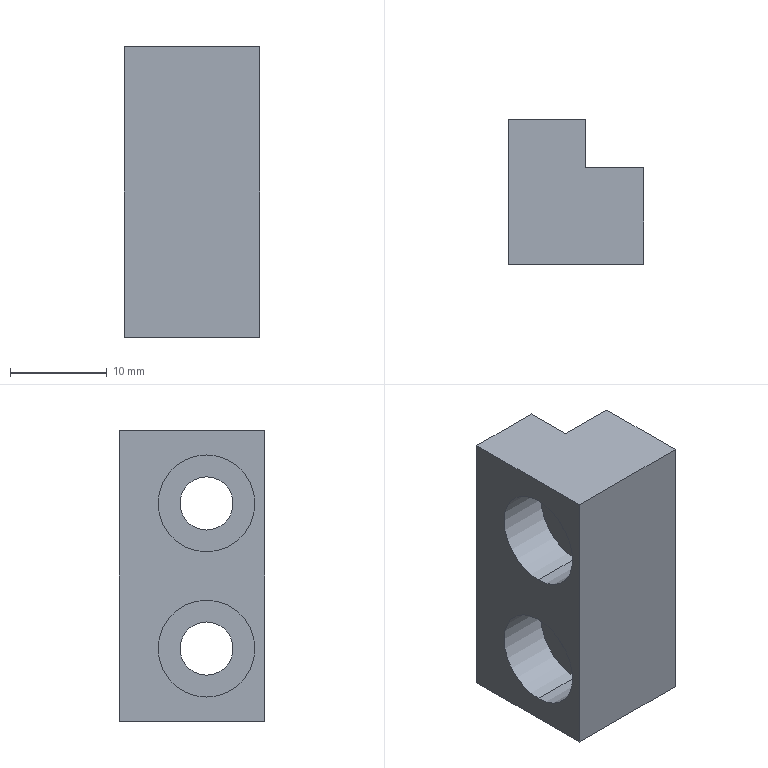Component | SolidWorks | 8TC-A15004-60-34B-1 | 1 solid | 18 faces | box 14 x 15 x 30 mm | volume 4143 mm3 | plane 10 | cylinder 8 | commonest cylinder face diameters 10 x4 5.5 x4 | material #45
build123d program:
from build123d import *

# Parameters (mm, degrees)
SKETCH1_W                                       = 15
SKETCH1_H                                       = 30
BOSS_EXTRUDE1_DEPTH                             = 7
SKETCH2_W                                       = 5
SKETCH2_H                                       = 6
CUT_EXTRUDE1_DEPTH                              = 32.706
M5_HEX_SOCKET_HEAD_CAP_SCREW_CBORE1_D           = 5.5
M5_HEX_SOCKET_HEAD_CAP_SCREW_CBORE1_CBORE_D     = 10
M5_HEX_SOCKET_HEAD_CAP_SCREW_CBORE1_CBORE_DEPTH = 5.4


with BuildPart() as part:
    # Sketch1 → Boss-Extrude1 (new, symmetric)
    with BuildSketch(Plane(origin=(0, 0, 0), x_dir=(1, 0, 0), z_dir=(0, 1, 0))):
        Rectangle(SKETCH1_W, SKETCH1_H)
    extrude(amount=BOSS_EXTRUDE1_DEPTH, both=True)

    # Sketch2 → Cut-Extrude1 (cut, through all)
    with BuildSketch(Plane.XY.offset(15)):
        with Locations((-5, -4)):
            Rectangle(SKETCH2_W, SKETCH2_H)
    extrude(amount=-CUT_EXTRUDE1_DEPTH, mode=Mode.SUBTRACT)

    # M5 Hex Socket Head Cap Screw CBORE1 (through all)
    with Locations(Plane(origin=(0, 7, 0), x_dir=(1, 0, 0), z_dir=(0, 1, 0))):
        with Locations((1.5, 7.5), (1.5, -7.5)):
            CounterBoreHole(M5_HEX_SOCKET_HEAD_CAP_SCREW_CBORE1_D / 2, M5_HEX_SOCKET_HEAD_CAP_SCREW_CBORE1_CBORE_D / 2, M5_HEX_SOCKET_HEAD_CAP_SCREW_CBORE1_CBORE_DEPTH)


solid = part.part

# Placed as in the assembly
solid = solid.moved(Location((-104.286, -69.5, 0), (180, 0, 90)))
STEP:
#1=COLOUR_RGB('',0.7922,0.8196,0.9333);
#2=FILL_AREA_STYLE_COLOUR('',#1);
#3=FILL_AREA_STYLE('',(#2));
#4=SURFACE_STYLE_FILL_AREA(#3);
#5=SURFACE_SIDE_STYLE('',(#4));
#6=SURFACE_STYLE_USAGE(.BOTH.,#5);
#7=PRESENTATION_STYLE_ASSIGNMENT((#6));
#8=CARTESIAN_POINT('',(-4.169,-2.795,0.4921));
#9=VERTEX_POINT('',#8);
#10=CARTESIAN_POINT('',(-4.169,-2.795,0.09843));
#11=VERTEX_POINT('',#10);
#12=CARTESIAN_POINT('',(-4.169,-2.795,0.2953));
#13=DIRECTION('',(-1.,0.,0.));
#14=DIRECTION('',(0.,0.,-1.));
#15=AXIS2_PLACEMENT_3D('',#12,#13,#14);
#16=CIRCLE('',#15,0.1969);
#17=EDGE_CURVE('',#9,#11,#16,.T.);
#18=ORIENTED_EDGE('',*,*,#17,.F.);
#19=CARTESIAN_POINT('',(-4.381,-2.795,0.4921));
#20=VERTEX_POINT('',#19);
#21=CARTESIAN_POINT('',(-4.381,-2.795,0.4921));
#22=DIRECTION('',(-1.,0.,0.));
#23=VECTOR('',#22,39.37);
#24=LINE('',#21,#23);
#25=EDGE_CURVE('',#9,#20,#24,.T.);
#26=ORIENTED_EDGE('',*,*,#25,.T.);
#27=CARTESIAN_POINT('',(-4.381,-2.795,0.09843));
#28=VERTEX_POINT('',#27);
#29=CARTESIAN_POINT('',(-4.381,-2.795,0.2953));
#30=DIRECTION('',(-1.,0.,0.));
#31=DIRECTION('',(0.,0.,-1.));
#32=AXIS2_PLACEMENT_3D('',#29,#30,#31);
#33=CIRCLE('',#32,0.1969);
#34=EDGE_CURVE('',#20,#28,#33,.T.);
#35=ORIENTED_EDGE('',*,*,#34,.T.);
#36=CARTESIAN_POINT('',(-4.381,-2.795,0.09843));
#37=DIRECTION('',(-1.,0.,0.));
#38=VECTOR('',#37,39.37);
#39=LINE('',#36,#38);
#40=EDGE_CURVE('',#11,#28,#39,.T.);
#41=ORIENTED_EDGE('',*,*,#40,.F.);
#42=EDGE_LOOP('',(#18,#26,#35,#41));
#43=FACE_OUTER_BOUND('',#42,.T.);
#44=CARTESIAN_POINT('',(-4.381,-2.795,0.2953));
#45=DIRECTION('',(-1.,0.,0.));
#46=DIRECTION('',(0.,0.,-1.));
#47=AXIS2_PLACEMENT_3D('',#44,#45,#46);
#48=CYLINDRICAL_SURFACE('',#47,0.1969);
#49=ADVANCED_FACE('',(#43),#48,.F.);
#50=CARTESIAN_POINT('',(-3.83,-2.795,0.4035));
#51=VERTEX_POINT('',#50);
#52=CARTESIAN_POINT('',(-3.83,-2.795,0.187));
#53=VERTEX_POINT('',#52);
#54=CARTESIAN_POINT('',(-3.83,-2.795,0.2953));
#55=DIRECTION('',(-1.,0.,0.));
#56=DIRECTION('',(0.,0.,-1.));
#57=AXIS2_PLACEMENT_3D('',#54,#55,#56);
#58=CIRCLE('',#57,0.1083);
#59=EDGE_CURVE('',#51,#53,#58,.T.);
#60=ORIENTED_EDGE('',*,*,#59,.F.);
#61=CARTESIAN_POINT('',(-4.169,-2.795,0.4035));
#62=VERTEX_POINT('',#61);
#63=CARTESIAN_POINT('',(-4.381,-2.795,0.4035));
#64=DIRECTION('',(-1.,0.,0.));
#65=VECTOR('',#64,39.37);
#66=LINE('',#63,#65);
#67=EDGE_CURVE('',#51,#62,#66,.T.);
#68=ORIENTED_EDGE('',*,*,#67,.T.);
#69=CARTESIAN_POINT('',(-4.169,-2.795,0.187));
#70=VERTEX_POINT('',#69);
#71=CARTESIAN_POINT('',(-4.169,-2.795,0.2953));
#72=DIRECTION('',(-1.,0.,0.));
#73=DIRECTION('',(0.,0.,-1.));
#74=AXIS2_PLACEMENT_3D('',#71,#72,#73);
#75=CIRCLE('',#74,0.1083);
#76=EDGE_CURVE('',#62,#70,#75,.T.);
#77=ORIENTED_EDGE('',*,*,#76,.T.);
#78=CARTESIAN_POINT('',(-4.381,-2.795,0.187));
#79=DIRECTION('',(-1.,0.,0.));
#80=VECTOR('',#79,39.37);
#81=LINE('',#78,#80);
#82=EDGE_CURVE('',#53,#70,#81,.T.);
#83=ORIENTED_EDGE('',*,*,#82,.F.);
#84=EDGE_LOOP('',(#60,#68,#77,#83));
#85=FACE_OUTER_BOUND('',#84,.T.);
#86=CARTESIAN_POINT('',(-4.381,-2.795,0.2953));
#87=DIRECTION('',(-1.,0.,0.));
#88=DIRECTION('',(0.,0.,-1.));
#89=AXIS2_PLACEMENT_3D('',#86,#87,#88);
#90=CYLINDRICAL_SURFACE('',#89,0.1083);
#91=ADVANCED_FACE('',(#85),#90,.F.);
#92=CARTESIAN_POINT('',(-4.169,-2.795,-0.09843));
#93=VERTEX_POINT('',#92);
#94=CARTESIAN_POINT('',(-4.169,-2.795,-0.4921));
#95=VERTEX_POINT('',#94);
#96=CARTESIAN_POINT('',(-4.169,-2.795,-0.2953));
#97=DIRECTION('',(-1.,0.,0.));
#98=DIRECTION('',(0.,0.,-1.));
#99=AXIS2_PLACEMENT_3D('',#96,#97,#98);
#100=CIRCLE('',#99,0.1969);
#101=EDGE_CURVE('',#93,#95,#100,.T.);
#102=ORIENTED_EDGE('',*,*,#101,.F.);
#103=CARTESIAN_POINT('',(-4.381,-2.795,-0.09843));
#104=VERTEX_POINT('',#103);
#105=CARTESIAN_POINT('',(-4.381,-2.795,-0.09843));
#106=DIRECTION('',(-1.,0.,0.));
#107=VECTOR('',#106,39.37);
#108=LINE('',#105,#107);
#109=EDGE_CURVE('',#93,#104,#108,.T.);
#110=ORIENTED_EDGE('',*,*,#109,.T.);
#111=CARTESIAN_POINT('',(-4.381,-2.795,-0.4921));
#112=VERTEX_POINT('',#111);
#113=CARTESIAN_POINT('',(-4.381,-2.795,-0.2953));
#114=DIRECTION('',(-1.,0.,0.));
#115=DIRECTION('',(0.,0.,-1.));
#116=AXIS2_PLACEMENT_3D('',#113,#114,#115);
#117=CIRCLE('',#116,0.1969);
#118=EDGE_CURVE('',#104,#112,#117,.T.);
#119=ORIENTED_EDGE('',*,*,#118,.T.);
#120=CARTESIAN_POINT('',(-4.381,-2.795,-0.4921));
#121=DIRECTION('',(-1.,0.,0.));
#122=VECTOR('',#121,39.37);
#123=LINE('',#120,#122);
#124=EDGE_CURVE('',#95,#112,#123,.T.);
#125=ORIENTED_EDGE('',*,*,#124,.F.);
#126=EDGE_LOOP('',(#102,#110,#119,#125));
#127=FACE_OUTER_BOUND('',#126,.T.);
#128=CARTESIAN_POINT('',(-4.381,-2.795,-0.2953));
#129=DIRECTION('',(-1.,0.,0.));
#130=DIRECTION('',(0.,0.,-1.));
#131=AXIS2_PLACEMENT_3D('',#128,#129,#130);
#132=CYLINDRICAL_SURFACE('',#131,0.1969);
#133=ADVANCED_FACE('',(#127),#132,.F.);
#134=CARTESIAN_POINT('',(-3.83,-2.795,-0.187));
#135=VERTEX_POINT('',#134);
#136=CARTESIAN_POINT('',(-3.83,-2.795,-0.4035));
#137=VERTEX_POINT('',#136);
#138=CARTESIAN_POINT('',(-3.83,-2.795,-0.2953));
#139=DIRECTION('',(-1.,0.,0.));
#140=DIRECTION('',(0.,0.,-1.));
#141=AXIS2_PLACEMENT_3D('',#138,#139,#140);
#142=CIRCLE('',#141,0.1083);
#143=EDGE_CURVE('',#135,#137,#142,.T.);
#144=ORIENTED_EDGE('',*,*,#143,.F.);
#145=CARTESIAN_POINT('',(-4.169,-2.795,-0.187));
#146=VERTEX_POINT('',#145);
#147=CARTESIAN_POINT('',(-4.381,-2.795,-0.187));
#148=DIRECTION('',(-1.,0.,0.));
#149=VECTOR('',#148,39.37);
#150=LINE('',#147,#149);
#151=EDGE_CURVE('',#135,#146,#150,.T.);
#152=ORIENTED_EDGE('',*,*,#151,.T.);
#153=CARTESIAN_POINT('',(-4.169,-2.795,-0.4035));
#154=VERTEX_POINT('',#153);
#155=CARTESIAN_POINT('',(-4.169,-2.795,-0.2953));
#156=DIRECTION('',(-1.,0.,0.));
#157=DIRECTION('',(0.,0.,-1.));
#158=AXIS2_PLACEMENT_3D('',#155,#156,#157);
#159=CIRCLE('',#158,0.1083);
#160=EDGE_CURVE('',#146,#154,#159,.T.);
#161=ORIENTED_EDGE('',*,*,#160,.T.);
#162=CARTESIAN_POINT('',(-4.381,-2.795,-0.4035));
#163=DIRECTION('',(-1.,0.,0.));
#164=VECTOR('',#163,39.37);
#165=LINE('',#162,#164);
#166=EDGE_CURVE('',#137,#154,#165,.T.);
#167=ORIENTED_EDGE('',*,*,#166,.F.);
#168=EDGE_LOOP('',(#144,#152,#161,#167));
#169=FACE_OUTER_BOUND('',#168,.T.);
#170=CARTESIAN_POINT('',(-4.381,-2.795,-0.2953));
#171=DIRECTION('',(-1.,0.,0.));
#172=DIRECTION('',(0.,0.,-1.));
#173=AXIS2_PLACEMENT_3D('',#170,#171,#172);
#174=CYLINDRICAL_SURFACE('',#173,0.1083);
#175=ADVANCED_FACE('',(#169),#174,.F.);
#176=CARTESIAN_POINT('',(-3.83,-2.638,0.5906));
#177=VERTEX_POINT('',#176);
#178=CARTESIAN_POINT('',(-3.83,-2.638,-0.5906));
#179=VERTEX_POINT('',#178);
#180=CARTESIAN_POINT('',(-3.83,-2.638,0.5906));
#181=DIRECTION('',(-0.,-0.,-1.));
#182=VECTOR('',#181,39.37);
#183=LINE('',#180,#182);
#184=EDGE_CURVE('',#177,#179,#183,.T.);
#185=ORIENTED_EDGE('',*,*,#184,.F.);
#186=CARTESIAN_POINT('',(-3.83,-3.031,0.5906));
#187=VERTEX_POINT('',#186);
#188=CARTESIAN_POINT('',(-3.83,-2.441,0.5906));
#189=DIRECTION('',(0.,1.,-0.));
#190=VECTOR('',#189,39.37);
#191=LINE('',#188,#190);
#192=EDGE_CURVE('',#187,#177,#191,.T.);
#193=ORIENTED_EDGE('',*,*,#192,.F.);
#194=CARTESIAN_POINT('',(-3.83,-3.031,-0.5906));
#195=VERTEX_POINT('',#194);
#196=CARTESIAN_POINT('',(-3.83,-3.031,-0.5906));
#197=DIRECTION('',(0.,0.,1.));
#198=VECTOR('',#197,39.37);
#199=LINE('',#196,#198);
#200=EDGE_CURVE('',#195,#187,#199,.T.);
#201=ORIENTED_EDGE('',*,*,#200,.F.);
#202=CARTESIAN_POINT('',(-3.83,-2.441,-0.5906));
#203=DIRECTION('',(-0.,-1.,0.));
#204=VECTOR('',#203,39.37);
#205=LINE('',#202,#204);
#206=EDGE_CURVE('',#179,#195,#205,.T.);
#207=ORIENTED_EDGE('',*,*,#206,.F.);
#208=EDGE_LOOP('',(#185,#193,#201,#207));
#209=FACE_OUTER_BOUND('',#208,.T.);
#210=CARTESIAN_POINT('',(-3.83,-2.795,-0.2953));
#211=DIRECTION('',(-1.,0.,0.));
#212=DIRECTION('',(0.,0.,-1.));
#213=AXIS2_PLACEMENT_3D('',#210,#211,#212);
#214=CIRCLE('',#213,0.1083);
#215=EDGE_CURVE('',#137,#135,#214,.T.);
#216=ORIENTED_EDGE('',*,*,#215,.T.);
#217=ORIENTED_EDGE('',*,*,#143,.T.);
#218=EDGE_LOOP('',(#216,#217));
#219=FACE_BOUND('',#218,.T.);
#220=CARTESIAN_POINT('',(-3.83,-2.795,0.2953));
#221=DIRECTION('',(-1.,0.,0.));
#222=DIRECTION('',(0.,0.,-1.));
#223=AXIS2_PLACEMENT_3D('',#220,#221,#222);
#224=CIRCLE('',#223,0.1083);
#225=EDGE_CURVE('',#53,#51,#224,.T.);
#226=ORIENTED_EDGE('',*,*,#225,.T.);
#227=ORIENTED_EDGE('',*,*,#59,.T.);
#228=EDGE_LOOP('',(#226,#227));
#229=FACE_BOUND('',#228,.T.);
#230=CARTESIAN_POINT('',(-3.83,-2.736,-0.));
#231=DIRECTION('',(1.,-0.,-0.));
#232=DIRECTION('',(0.,0.,1.));
#233=AXIS2_PLACEMENT_3D('',#230,#231,#232);
#234=PLANE('',#233);
#235=ADVANCED_FACE('',(#209,#219,#229),#234,.T.);
#236=ORIENTED_EDGE('',*,*,#200,.T.);
#237=CARTESIAN_POINT('',(-4.381,-3.031,0.5906));
#238=VERTEX_POINT('',#237);
#239=CARTESIAN_POINT('',(-4.381,-3.031,0.5906));
#240=DIRECTION('',(1.,-0.,-0.));
#241=VECTOR('',#240,39.37);
#242=LINE('',#239,#241);
#243=EDGE_CURVE('',#238,#187,#242,.T.);
#244=ORIENTED_EDGE('',*,*,#243,.F.);
#245=CARTESIAN_POINT('',(-4.381,-3.031,-0.5906));
#246=VERTEX_POINT('',#245);
#247=CARTESIAN_POINT('',(-4.381,-3.031,-0.5906));
#248=DIRECTION('',(0.,0.,1.));
#249=VECTOR('',#248,39.37);
#250=LINE('',#247,#249);
#251=EDGE_CURVE('',#246,#238,#250,.T.);
#252=ORIENTED_EDGE('',*,*,#251,.F.);
#253=CARTESIAN_POINT('',(-4.381,-3.031,-0.5906));
#254=DIRECTION('',(1.,-0.,-0.));
#255=VECTOR('',#254,39.37);
#256=LINE('',#253,#255);
#257=EDGE_CURVE('',#246,#195,#256,.T.);
#258=ORIENTED_EDGE('',*,*,#257,.T.);
#259=EDGE_LOOP('',(#236,#244,#252,#258));
#260=FACE_OUTER_BOUND('',#259,.T.);
#261=CARTESIAN_POINT('',(-4.381,-3.031,-0.5906));
#262=DIRECTION('',(0.,1.,-0.));
#263=DIRECTION('',(-0.,-0.,-1.));
#264=AXIS2_PLACEMENT_3D('',#261,#262,#263);
#265=PLANE('',#264);
#266=ADVANCED_FACE('',(#260),#265,.F.);
#267=CARTESIAN_POINT('',(-4.066,-2.638,0.5906));
#268=VERTEX_POINT('',#267);
#269=CARTESIAN_POINT('',(-3.83,-2.638,0.5906));
#270=DIRECTION('',(-1.,0.,0.));
#271=VECTOR('',#270,39.37);
#272=LINE('',#269,#271);
#273=EDGE_CURVE('',#177,#268,#272,.T.);
#274=ORIENTED_EDGE('',*,*,#273,.T.);
#275=CARTESIAN_POINT('',(-4.066,-2.441,0.5906));
#276=VERTEX_POINT('',#275);
#277=CARTESIAN_POINT('',(-4.066,-2.441,0.5906));
#278=DIRECTION('',(0.,1.,-0.));
#279=VECTOR('',#278,39.37);
#280=LINE('',#277,#279);
#281=EDGE_CURVE('',#268,#276,#280,.T.);
#282=ORIENTED_EDGE('',*,*,#281,.T.);
#283=CARTESIAN_POINT('',(-4.381,-2.441,0.5906));
#284=VERTEX_POINT('',#283);
#285=CARTESIAN_POINT('',(-4.381,-2.441,0.5906));
#286=DIRECTION('',(1.,-0.,-0.));
#287=VECTOR('',#286,39.37);
#288=LINE('',#285,#287);
#289=EDGE_CURVE('',#284,#276,#288,.T.);
#290=ORIENTED_EDGE('',*,*,#289,.F.);
#291=CARTESIAN_POINT('',(-4.381,-2.441,0.5906));
#292=DIRECTION('',(0.,1.,-0.));
#293=VECTOR('',#292,39.37);
#294=LINE('',#291,#293);
#295=EDGE_CURVE('',#238,#284,#294,.T.);
#296=ORIENTED_EDGE('',*,*,#295,.F.);
#297=ORIENTED_EDGE('',*,*,#243,.T.);
#298=ORIENTED_EDGE('',*,*,#192,.T.);
#299=EDGE_LOOP('',(#274,#282,#290,#296,#297,#298));
#300=FACE_OUTER_BOUND('',#299,.T.);
#301=CARTESIAN_POINT('',(-4.381,-2.441,0.5906));
#302=DIRECTION('',(-0.,-0.,-1.));
#303=DIRECTION('',(-0.,-1.,0.));
#304=AXIS2_PLACEMENT_3D('',#301,#302,#303);
#305=PLANE('',#304);
#306=ADVANCED_FACE('',(#300),#305,.F.);
#307=ORIENTED_EDGE('',*,*,#289,.T.);
#308=CARTESIAN_POINT('',(-4.066,-2.441,-0.5906));
#309=VERTEX_POINT('',#308);
#310=CARTESIAN_POINT('',(-4.066,-2.441,0.5906));
#311=DIRECTION('',(-0.,-0.,-1.));
#312=VECTOR('',#311,39.37);
#313=LINE('',#310,#312);
#314=EDGE_CURVE('',#276,#309,#313,.T.);
#315=ORIENTED_EDGE('',*,*,#314,.T.);
#316=CARTESIAN_POINT('',(-4.381,-2.441,-0.5906));
#317=VERTEX_POINT('',#316);
#318=CARTESIAN_POINT('',(-4.381,-2.441,-0.5906));
#319=DIRECTION('',(1.,-0.,-0.));
#320=VECTOR('',#319,39.37);
#321=LINE('',#318,#320);
#322=EDGE_CURVE('',#317,#309,#321,.T.);
#323=ORIENTED_EDGE('',*,*,#322,.F.);
#324=CARTESIAN_POINT('',(-4.381,-2.441,-0.5906));
#325=DIRECTION('',(-0.,-0.,-1.));
#326=VECTOR('',#325,39.37);
#327=LINE('',#324,#326);
#328=EDGE_CURVE('',#284,#317,#327,.T.);
#329=ORIENTED_EDGE('',*,*,#328,.F.);
#330=EDGE_LOOP('',(#307,#315,#323,#329));
#331=FACE_OUTER_BOUND('',#330,.T.);
#332=CARTESIAN_POINT('',(-4.381,-2.441,-0.5906));
#333=DIRECTION('',(-0.,-1.,0.));
#334=DIRECTION('',(0.,0.,1.));
#335=AXIS2_PLACEMENT_3D('',#332,#333,#334);
#336=PLANE('',#335);
#337=ADVANCED_FACE('',(#331),#336,.F.);
#338=ORIENTED_EDGE('',*,*,#322,.T.);
#339=CARTESIAN_POINT('',(-4.066,-2.638,-0.5906));
#340=VERTEX_POINT('',#339);
#341=CARTESIAN_POINT('',(-4.066,-2.441,-0.5906));
#342=DIRECTION('',(0.,1.,-0.));
#343=VECTOR('',#342,39.37);
#344=LINE('',#341,#343);
#345=EDGE_CURVE('',#340,#309,#344,.T.);
#346=ORIENTED_EDGE('',*,*,#345,.F.);
#347=CARTESIAN_POINT('',(-3.83,-2.638,-0.5906));
#348=DIRECTION('',(-1.,0.,0.));
#349=VECTOR('',#348,39.37);
#350=LINE('',#347,#349);
#351=EDGE_CURVE('',#179,#340,#350,.T.);
#352=ORIENTED_EDGE('',*,*,#351,.F.);
#353=ORIENTED_EDGE('',*,*,#206,.T.);
#354=ORIENTED_EDGE('',*,*,#257,.F.);
#355=CARTESIAN_POINT('',(-4.381,-2.441,-0.5906));
#356=DIRECTION('',(-0.,-1.,0.));
#357=VECTOR('',#356,39.37);
#358=LINE('',#355,#357);
#359=EDGE_CURVE('',#317,#246,#358,.T.);
#360=ORIENTED_EDGE('',*,*,#359,.F.);
#361=EDGE_LOOP('',(#338,#346,#352,#353,#354,#360));
#362=FACE_OUTER_BOUND('',#361,.T.);
#363=CARTESIAN_POINT('',(-4.381,-2.441,-0.5906));
#364=DIRECTION('',(0.,0.,1.));
#365=DIRECTION('',(0.,1.,-0.));
#366=AXIS2_PLACEMENT_3D('',#363,#364,#365);
#367=PLANE('',#366);
#368=ADVANCED_FACE('',(#362),#367,.F.);
#369=CARTESIAN_POINT('',(-4.381,-2.795,0.2953));
#370=DIRECTION('',(-1.,0.,0.));
#371=DIRECTION('',(0.,0.,-1.));
#372=AXIS2_PLACEMENT_3D('',#369,#370,#371);
#373=CIRCLE('',#372,0.1969);
#374=EDGE_CURVE('',#28,#20,#373,.T.);
#375=ORIENTED_EDGE('',*,*,#374,.F.);
#376=ORIENTED_EDGE('',*,*,#34,.F.);
#377=EDGE_LOOP('',(#375,#376));
#378=FACE_BOUND('',#377,.T.);
#379=CARTESIAN_POINT('',(-4.381,-2.795,-0.2953));
#380=DIRECTION('',(-1.,0.,0.));
#381=DIRECTION('',(0.,0.,-1.));
#382=AXIS2_PLACEMENT_3D('',#379,#380,#381);
#383=CIRCLE('',#382,0.1969);
#384=EDGE_CURVE('',#112,#104,#383,.T.);
#385=ORIENTED_EDGE('',*,*,#384,.F.);
#386=ORIENTED_EDGE('',*,*,#118,.F.);
#387=EDGE_LOOP('',(#385,#386));
#388=FACE_BOUND('',#387,.T.);
#389=ORIENTED_EDGE('',*,*,#251,.T.);
#390=ORIENTED_EDGE('',*,*,#295,.T.);
#391=ORIENTED_EDGE('',*,*,#328,.T.);
#392=ORIENTED_EDGE('',*,*,#359,.T.);
#393=EDGE_LOOP('',(#389,#390,#391,#392));
#394=FACE_OUTER_BOUND('',#393,.T.);
#395=CARTESIAN_POINT('',(-4.381,-2.736,-0.));
#396=DIRECTION('',(1.,-0.,-0.));
#397=DIRECTION('',(0.,0.,1.));
#398=AXIS2_PLACEMENT_3D('',#395,#396,#397);
#399=PLANE('',#398);
#400=ADVANCED_FACE('',(#378,#388,#394),#399,.F.);
#401=ORIENTED_EDGE('',*,*,#345,.T.);
#402=ORIENTED_EDGE('',*,*,#314,.F.);
#403=ORIENTED_EDGE('',*,*,#281,.F.);
#404=CARTESIAN_POINT('',(-4.066,-2.638,0.5906));
#405=DIRECTION('',(-0.,-0.,-1.));
#406=VECTOR('',#405,39.37);
#407=LINE('',#404,#406);
#408=EDGE_CURVE('',#268,#340,#407,.T.);
#409=ORIENTED_EDGE('',*,*,#408,.T.);
#410=EDGE_LOOP('',(#401,#402,#403,#409));
#411=FACE_OUTER_BOUND('',#410,.T.);
#412=CARTESIAN_POINT('',(-4.066,-2.441,0.5906));
#413=DIRECTION('',(-1.,0.,0.));
#414=DIRECTION('',(-0.,-0.,-1.));
#415=AXIS2_PLACEMENT_3D('',#412,#413,#414);
#416=PLANE('',#415);
#417=ADVANCED_FACE('',(#411),#416,.F.);
#418=ORIENTED_EDGE('',*,*,#351,.T.);
#419=ORIENTED_EDGE('',*,*,#408,.F.);
#420=ORIENTED_EDGE('',*,*,#273,.F.);
#421=ORIENTED_EDGE('',*,*,#184,.T.);
#422=EDGE_LOOP('',(#418,#419,#420,#421));
#423=FACE_OUTER_BOUND('',#422,.T.);
#424=CARTESIAN_POINT('',(-3.83,-2.638,0.5906));
#425=DIRECTION('',(-0.,-1.,0.));
#426=DIRECTION('',(0.,0.,1.));
#427=AXIS2_PLACEMENT_3D('',#424,#425,#426);
#428=PLANE('',#427);
#429=ADVANCED_FACE('',(#423),#428,.F.);
#430=ORIENTED_EDGE('',*,*,#151,.F.);
#431=ORIENTED_EDGE('',*,*,#215,.F.);
#432=ORIENTED_EDGE('',*,*,#166,.T.);
#433=CARTESIAN_POINT('',(-4.169,-2.795,-0.2953));
#434=DIRECTION('',(-1.,0.,0.));
#435=DIRECTION('',(0.,0.,-1.));
#436=AXIS2_PLACEMENT_3D('',#433,#434,#435);
#437=CIRCLE('',#436,0.1083);
#438=EDGE_CURVE('',#154,#146,#437,.T.);
#439=ORIENTED_EDGE('',*,*,#438,.T.);
#440=EDGE_LOOP('',(#430,#431,#432,#439));
#441=FACE_OUTER_BOUND('',#440,.T.);
#442=CARTESIAN_POINT('',(-4.381,-2.795,-0.2953));
#443=DIRECTION('',(-1.,0.,0.));
#444=DIRECTION('',(0.,0.,-1.));
#445=AXIS2_PLACEMENT_3D('',#442,#443,#444);
#446=CYLINDRICAL_SURFACE('',#445,0.1083);
#447=ADVANCED_FACE('',(#441),#446,.F.);
#448=ORIENTED_EDGE('',*,*,#438,.F.);
#449=ORIENTED_EDGE('',*,*,#160,.F.);
#450=EDGE_LOOP('',(#448,#449));
#451=FACE_BOUND('',#450,.T.);
#452=CARTESIAN_POINT('',(-4.169,-2.795,-0.2953));
#453=DIRECTION('',(-1.,0.,0.));
#454=DIRECTION('',(0.,0.,-1.));
#455=AXIS2_PLACEMENT_3D('',#452,#453,#454);
#456=CIRCLE('',#455,0.1969);
#457=EDGE_CURVE('',#95,#93,#456,.T.);
#458=ORIENTED_EDGE('',*,*,#457,.T.);
#459=ORIENTED_EDGE('',*,*,#101,.T.);
#460=EDGE_LOOP('',(#458,#459));
#461=FACE_OUTER_BOUND('',#460,.T.);
#462=CARTESIAN_POINT('',(-4.169,-2.904,-0.2953));
#463=DIRECTION('',(1.,-0.,-0.));
#464=DIRECTION('',(0.,0.,1.));
#465=AXIS2_PLACEMENT_3D('',#462,#463,#464);
#466=PLANE('',#465);
#467=ADVANCED_FACE('',(#451,#461),#466,.F.);
#468=ORIENTED_EDGE('',*,*,#109,.F.);
#469=ORIENTED_EDGE('',*,*,#457,.F.);
#470=ORIENTED_EDGE('',*,*,#124,.T.);
#471=ORIENTED_EDGE('',*,*,#384,.T.);
#472=EDGE_LOOP('',(#468,#469,#470,#471));
#473=FACE_OUTER_BOUND('',#472,.T.);
#474=CARTESIAN_POINT('',(-4.381,-2.795,-0.2953));
#475=DIRECTION('',(-1.,0.,0.));
#476=DIRECTION('',(0.,0.,-1.));
#477=AXIS2_PLACEMENT_3D('',#474,#475,#476);
#478=CYLINDRICAL_SURFACE('',#477,0.1969);
#479=ADVANCED_FACE('',(#473),#478,.F.);
#480=ORIENTED_EDGE('',*,*,#67,.F.);
#481=ORIENTED_EDGE('',*,*,#225,.F.);
#482=ORIENTED_EDGE('',*,*,#82,.T.);
#483=CARTESIAN_POINT('',(-4.169,-2.795,0.2953));
#484=DIRECTION('',(-1.,0.,0.));
#485=DIRECTION('',(0.,0.,-1.));
#486=AXIS2_PLACEMENT_3D('',#483,#484,#485);
#487=CIRCLE('',#486,0.1083);
#488=EDGE_CURVE('',#70,#62,#487,.T.);
#489=ORIENTED_EDGE('',*,*,#488,.T.);
#490=EDGE_LOOP('',(#480,#481,#482,#489));
#491=FACE_OUTER_BOUND('',#490,.T.);
#492=CARTESIAN_POINT('',(-4.381,-2.795,0.2953));
#493=DIRECTION('',(-1.,0.,0.));
#494=DIRECTION('',(0.,0.,-1.));
#495=AXIS2_PLACEMENT_3D('',#492,#493,#494);
#496=CYLINDRICAL_SURFACE('',#495,0.1083);
#497=ADVANCED_FACE('',(#491),#496,.F.);
#498=ORIENTED_EDGE('',*,*,#488,.F.);
#499=ORIENTED_EDGE('',*,*,#76,.F.);
#500=EDGE_LOOP('',(#498,#499));
#501=FACE_BOUND('',#500,.T.);
#502=CARTESIAN_POINT('',(-4.169,-2.795,0.2953));
#503=DIRECTION('',(-1.,0.,0.));
#504=DIRECTION('',(0.,0.,-1.));
#505=AXIS2_PLACEMENT_3D('',#502,#503,#504);
#506=CIRCLE('',#505,0.1969);
#507=EDGE_CURVE('',#11,#9,#506,.T.);
#508=ORIENTED_EDGE('',*,*,#507,.T.);
#509=ORIENTED_EDGE('',*,*,#17,.T.);
#510=EDGE_LOOP('',(#508,#509));
#511=FACE_OUTER_BOUND('',#510,.T.);
#512=CARTESIAN_POINT('',(-4.169,-2.904,0.2953));
#513=DIRECTION('',(1.,-0.,-0.));
#514=DIRECTION('',(0.,0.,1.));
#515=AXIS2_PLACEMENT_3D('',#512,#513,#514);
#516=PLANE('',#515);
#517=ADVANCED_FACE('',(#501,#511),#516,.F.);
#518=ORIENTED_EDGE('',*,*,#25,.F.);
#519=ORIENTED_EDGE('',*,*,#507,.F.);
#520=ORIENTED_EDGE('',*,*,#40,.T.);
#521=ORIENTED_EDGE('',*,*,#374,.T.);
#522=EDGE_LOOP('',(#518,#519,#520,#521));
#523=FACE_OUTER_BOUND('',#522,.T.);
#524=CARTESIAN_POINT('',(-4.381,-2.795,0.2953));
#525=DIRECTION('',(-1.,0.,0.));
#526=DIRECTION('',(0.,0.,-1.));
#527=AXIS2_PLACEMENT_3D('',#524,#525,#526);
#528=CYLINDRICAL_SURFACE('',#527,0.1969);
#529=ADVANCED_FACE('',(#523),#528,.F.);
#530=CLOSED_SHELL('',(#49,#91,#133,#175,#235,#266,#306,#337,#368,#400,#417,#429,#447,#467,#479,#497,#517,#529));
#531=MANIFOLD_SOLID_BREP('',#530);
#532=STYLED_ITEM('',(#7),#531);
#533=PRESENTATION_LAYER_ASSIGNMENT('','',(#532));
#534=CARTESIAN_POINT('',(0.,0.,0.));
#535=DIRECTION('',(0.,0.,1.));
#536=DIRECTION('',(1.,0.,0.));
#537=AXIS2_PLACEMENT_3D('',#534,#535,#536);
#538=(LENGTH_UNIT()NAMED_UNIT(*)SI_UNIT($,.METRE.));
#539=LENGTH_MEASURE_WITH_UNIT(LENGTH_MEASURE(0.0254),#538);
#540=DIMENSIONAL_EXPONENTS(1.,0.,0.,0.,0.,0.,0.);
#541=(CONVERSION_BASED_UNIT('',#539)LENGTH_UNIT()NAMED_UNIT(#540));
#542=UNCERTAINTY_MEASURE_WITH_UNIT(LENGTH_MEASURE(0.00001),#541,'','');
#543=(NAMED_UNIT(*)PLANE_ANGLE_UNIT()SI_UNIT($,.RADIAN.));
#544=(NAMED_UNIT(*)SI_UNIT($,.STERADIAN.)SOLID_ANGLE_UNIT());
#545=(GEOMETRIC_REPRESENTATION_CONTEXT(3)GLOBAL_UNCERTAINTY_ASSIGNED_CONTEXT((#542))GLOBAL_UNIT_ASSIGNED_CONTEXT((#541,#543,#544))REPRESENTATION_CONTEXT('',''));
#546=ADVANCED_BREP_SHAPE_REPRESENTATION('',(#531,#537),#545);
#547=(LENGTH_UNIT()NAMED_UNIT(*)SI_UNIT($,.METRE.));
#548=LENGTH_MEASURE_WITH_UNIT(LENGTH_MEASURE(0.0254),#547);
#549=DIMENSIONAL_EXPONENTS(1.,0.,0.,0.,0.,0.,0.);
#550=(CONVERSION_BASED_UNIT('',#548)LENGTH_UNIT()NAMED_UNIT(#549));
#551=UNCERTAINTY_MEASURE_WITH_UNIT(LENGTH_MEASURE(0.00001),#550,'','');
#552=(NAMED_UNIT(*)PLANE_ANGLE_UNIT()SI_UNIT($,.RADIAN.));
#553=(NAMED_UNIT(*)SI_UNIT($,.STERADIAN.)SOLID_ANGLE_UNIT());
#554=(GEOMETRIC_REPRESENTATION_CONTEXT(3)GLOBAL_UNCERTAINTY_ASSIGNED_CONTEXT((#551))GLOBAL_UNIT_ASSIGNED_CONTEXT((#550,#552,#553))REPRESENTATION_CONTEXT('',''));
#555=MECHANICAL_DESIGN_GEOMETRIC_PRESENTATION_REPRESENTATION('',(#532),#554);